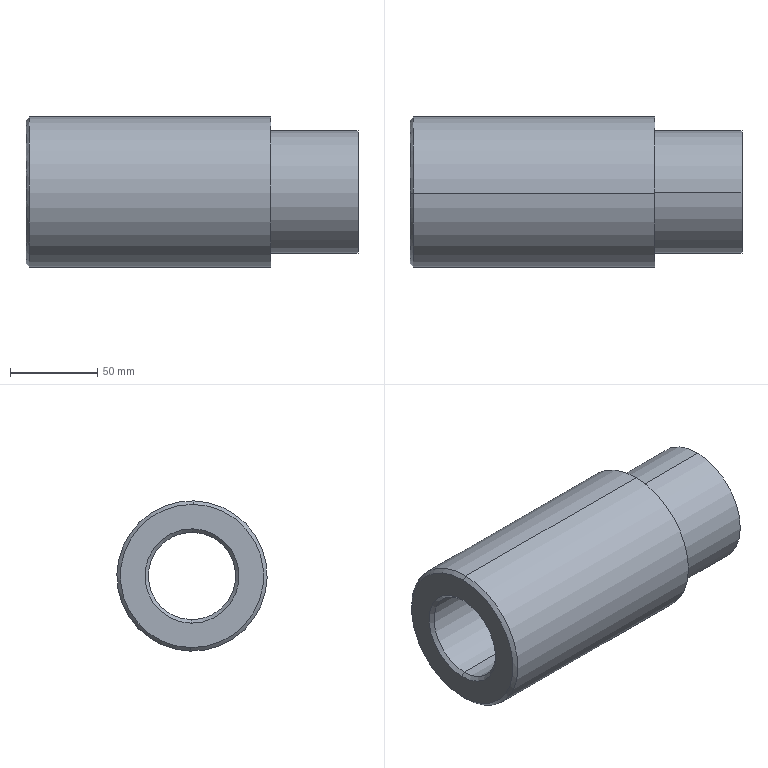Component | SolidWorks | 216InnerTubeAssembly-1_SpringSleeve-1 | 1 solid | 18 faces | box 190 x 86 x 86 mm | volume 501706 mm3 | cylinder 8 | cone 6 | plane 4 | commonest cylinder face diameters 86 x2 69.99 x2 60 x2 50 x2 | material Alloy Steel
build123d program:
from build123d import *


with BuildPart() as part:
    # Model → Revolve1 (revolve)
    with BuildSketch(Plane.XY, mode=Mode.PRIVATE) as revolve1_sk:
        Polygon((-150.007, 25), (-188.007, 25), (-190.007, 27), (-190.007, 41), (-188.007, 43), (-50.007, 43), (-50.007, 34.995), (-0.006987, 34.995), (-0.006987, 32), (-2.007, 30), (-150.007, 30), align=None)
    revolve(revolve1_sk.sketch.rotate(Axis((0, 0, 0), (-1, 0, 0)), 90), axis=Axis((0, 0, 0), (-1, 0, 0)))


solid = part.part

# Placed as in the assembly
solid = solid.moved(Location((322.098, 0, 0), (0, 0, 0)))
STEP:
#1=CARTESIAN_POINT('',(5.279,-0.01767,0.9841));
#2=VERTEX_POINT('',#1);
#3=CARTESIAN_POINT('',(5.279,0.01767,-0.9841));
#4=VERTEX_POINT('',#3);
#5=CARTESIAN_POINT('',(5.279,-0.,0.));
#6=DIRECTION('',(1.,0.,-0.));
#7=DIRECTION('',(0.,0.01796,-0.9998));
#8=AXIS2_PLACEMENT_3D('',#5,#6,#7);
#9=CIRCLE('',#8,0.9843);
#10=EDGE_CURVE('',#2,#4,#9,.T.);
#11=ORIENTED_EDGE('',*,*,#10,.T.);
#12=CARTESIAN_POINT('',(5.2,0.01909,-1.063));
#13=VERTEX_POINT('',#12);
#14=CARTESIAN_POINT('',(5.279,0.01767,-0.9841));
#15=DIRECTION('',(-0.7071,0.0127,-0.707));
#16=VECTOR('',#15,39.37);
#17=LINE('',#14,#16);
#18=EDGE_CURVE('',#4,#13,#17,.T.);
#19=ORIENTED_EDGE('',*,*,#18,.T.);
#20=CARTESIAN_POINT('',(5.2,-0.01909,1.063));
#21=VERTEX_POINT('',#20);
#22=CARTESIAN_POINT('',(5.2,-0.,0.));
#23=DIRECTION('',(1.,0.,-0.));
#24=DIRECTION('',(0.,0.01796,-0.9998));
#25=AXIS2_PLACEMENT_3D('',#22,#23,#24);
#26=CIRCLE('',#25,1.063);
#27=EDGE_CURVE('',#21,#13,#26,.T.);
#28=ORIENTED_EDGE('',*,*,#27,.F.);
#29=CARTESIAN_POINT('',(5.279,-0.01767,0.9841));
#30=DIRECTION('',(-0.7071,-0.0127,0.707));
#31=VECTOR('',#30,39.37);
#32=LINE('',#29,#31);
#33=EDGE_CURVE('',#2,#21,#32,.T.);
#34=ORIENTED_EDGE('',*,*,#33,.F.);
#35=EDGE_LOOP('',(#11,#19,#28,#34));
#36=FACE_OUTER_BOUND('',#35,.T.);
#37=CARTESIAN_POINT('',(5.279,-0.,0.));
#38=DIRECTION('',(-1.,-0.,0.));
#39=DIRECTION('',(0.,-0.01796,0.9998));
#40=AXIS2_PLACEMENT_3D('',#37,#38,#39);
#41=CONICAL_SURFACE('',#40,0.9843,0.7854);
#42=ADVANCED_FACE('',(#36),#41,.F.);
#43=CARTESIAN_POINT('',(5.2,0.02898,-1.614));
#44=VERTEX_POINT('',#43);
#45=CARTESIAN_POINT('',(5.2,-0.02898,1.614));
#46=VERTEX_POINT('',#45);
#47=CARTESIAN_POINT('',(5.2,-0.,0.));
#48=DIRECTION('',(1.,0.,-0.));
#49=DIRECTION('',(0.,0.01796,-0.9998));
#50=AXIS2_PLACEMENT_3D('',#47,#48,#49);
#51=CIRCLE('',#50,1.614);
#52=EDGE_CURVE('',#44,#46,#51,.T.);
#53=ORIENTED_EDGE('',*,*,#52,.T.);
#54=CARTESIAN_POINT('',(5.279,-0.0304,1.693));
#55=VERTEX_POINT('',#54);
#56=CARTESIAN_POINT('',(5.279,-0.0304,1.693));
#57=DIRECTION('',(0.7071,-0.0127,0.707));
#58=VECTOR('',#57,39.37);
#59=LINE('',#56,#58);
#60=EDGE_CURVE('',#46,#55,#59,.T.);
#61=ORIENTED_EDGE('',*,*,#60,.T.);
#62=CARTESIAN_POINT('',(5.279,0.0304,-1.693));
#63=VERTEX_POINT('',#62);
#64=CARTESIAN_POINT('',(5.279,-0.,0.));
#65=DIRECTION('',(1.,0.,-0.));
#66=DIRECTION('',(0.,0.01796,-0.9998));
#67=AXIS2_PLACEMENT_3D('',#64,#65,#66);
#68=CIRCLE('',#67,1.693);
#69=EDGE_CURVE('',#63,#55,#68,.T.);
#70=ORIENTED_EDGE('',*,*,#69,.F.);
#71=CARTESIAN_POINT('',(5.279,0.0304,-1.693));
#72=DIRECTION('',(0.7071,0.0127,-0.707));
#73=VECTOR('',#72,39.37);
#74=LINE('',#71,#73);
#75=EDGE_CURVE('',#44,#63,#74,.T.);
#76=ORIENTED_EDGE('',*,*,#75,.F.);
#77=EDGE_LOOP('',(#53,#61,#70,#76));
#78=FACE_OUTER_BOUND('',#77,.T.);
#79=CARTESIAN_POINT('',(5.279,-0.,0.));
#80=DIRECTION('',(1.,0.,-0.));
#81=DIRECTION('',(0.,0.01796,-0.9998));
#82=AXIS2_PLACEMENT_3D('',#79,#80,#81);
#83=CONICAL_SURFACE('',#82,1.693,0.7854);
#84=ADVANCED_FACE('',(#78),#83,.T.);
#85=ORIENTED_EDGE('',*,*,#69,.T.);
#86=CARTESIAN_POINT('',(10.712,-0.0304,1.693));
#87=VERTEX_POINT('',#86);
#88=CARTESIAN_POINT('',(12.681,-0.0304,1.693));
#89=DIRECTION('',(1.,0.,-0.));
#90=VECTOR('',#89,39.37);
#91=LINE('',#88,#90);
#92=EDGE_CURVE('',#55,#87,#91,.T.);
#93=ORIENTED_EDGE('',*,*,#92,.T.);
#94=CARTESIAN_POINT('',(10.712,0.0304,-1.693));
#95=VERTEX_POINT('',#94);
#96=CARTESIAN_POINT('',(10.712,-0.,0.));
#97=DIRECTION('',(1.,0.,-0.));
#98=DIRECTION('',(0.,0.01796,-0.9998));
#99=AXIS2_PLACEMENT_3D('',#96,#97,#98);
#100=CIRCLE('',#99,1.693);
#101=EDGE_CURVE('',#95,#87,#100,.T.);
#102=ORIENTED_EDGE('',*,*,#101,.F.);
#103=CARTESIAN_POINT('',(12.681,0.0304,-1.693));
#104=DIRECTION('',(1.,0.,-0.));
#105=VECTOR('',#104,39.37);
#106=LINE('',#103,#105);
#107=EDGE_CURVE('',#63,#95,#106,.T.);
#108=ORIENTED_EDGE('',*,*,#107,.F.);
#109=EDGE_LOOP('',(#85,#93,#102,#108));
#110=FACE_OUTER_BOUND('',#109,.T.);
#111=CARTESIAN_POINT('',(12.681,-0.,0.));
#112=DIRECTION('',(1.,0.,-0.));
#113=DIRECTION('',(0.,0.01796,-0.9998));
#114=AXIS2_PLACEMENT_3D('',#111,#112,#113);
#115=CYLINDRICAL_SURFACE('',#114,1.693);
#116=ADVANCED_FACE('',(#110),#115,.T.);
#117=CARTESIAN_POINT('',(10.712,0.02474,-1.378));
#118=VERTEX_POINT('',#117);
#119=CARTESIAN_POINT('',(10.712,-0.02474,1.378));
#120=VERTEX_POINT('',#119);
#121=CARTESIAN_POINT('',(10.712,-0.,0.));
#122=DIRECTION('',(1.,0.,-0.));
#123=DIRECTION('',(0.,0.01796,-0.9998));
#124=AXIS2_PLACEMENT_3D('',#121,#122,#123);
#125=CIRCLE('',#124,1.378);
#126=EDGE_CURVE('',#118,#120,#125,.T.);
#127=ORIENTED_EDGE('',*,*,#126,.T.);
#128=CARTESIAN_POINT('',(12.681,-0.02474,1.378));
#129=VERTEX_POINT('',#128);
#130=CARTESIAN_POINT('',(12.681,-0.02474,1.378));
#131=DIRECTION('',(1.,0.,-0.));
#132=VECTOR('',#131,39.37);
#133=LINE('',#130,#132);
#134=EDGE_CURVE('',#120,#129,#133,.T.);
#135=ORIENTED_EDGE('',*,*,#134,.T.);
#136=CARTESIAN_POINT('',(12.681,0.02474,-1.378));
#137=VERTEX_POINT('',#136);
#138=CARTESIAN_POINT('',(12.681,-0.,0.));
#139=DIRECTION('',(1.,0.,-0.));
#140=DIRECTION('',(0.,0.01796,-0.9998));
#141=AXIS2_PLACEMENT_3D('',#138,#139,#140);
#142=CIRCLE('',#141,1.378);
#143=EDGE_CURVE('',#137,#129,#142,.T.);
#144=ORIENTED_EDGE('',*,*,#143,.F.);
#145=CARTESIAN_POINT('',(12.681,0.02474,-1.378));
#146=DIRECTION('',(1.,0.,-0.));
#147=VECTOR('',#146,39.37);
#148=LINE('',#145,#147);
#149=EDGE_CURVE('',#118,#137,#148,.T.);
#150=ORIENTED_EDGE('',*,*,#149,.F.);
#151=EDGE_LOOP('',(#127,#135,#144,#150));
#152=FACE_OUTER_BOUND('',#151,.T.);
#153=CARTESIAN_POINT('',(12.681,-0.,0.));
#154=DIRECTION('',(1.,0.,-0.));
#155=DIRECTION('',(0.,0.01796,-0.9998));
#156=AXIS2_PLACEMENT_3D('',#153,#154,#155);
#157=CYLINDRICAL_SURFACE('',#156,1.378);
#158=ADVANCED_FACE('',(#152),#157,.T.);
#159=CARTESIAN_POINT('',(12.602,-0.02121,1.181));
#160=VERTEX_POINT('',#159);
#161=CARTESIAN_POINT('',(12.602,0.02121,-1.181));
#162=VERTEX_POINT('',#161);
#163=CARTESIAN_POINT('',(12.602,-0.,0.));
#164=DIRECTION('',(1.,0.,-0.));
#165=DIRECTION('',(0.,0.01796,-0.9998));
#166=AXIS2_PLACEMENT_3D('',#163,#164,#165);
#167=CIRCLE('',#166,1.181);
#168=EDGE_CURVE('',#160,#162,#167,.T.);
#169=ORIENTED_EDGE('',*,*,#168,.F.);
#170=CARTESIAN_POINT('',(12.681,-0.02262,1.26));
#171=VERTEX_POINT('',#170);
#172=CARTESIAN_POINT('',(12.681,-0.02262,1.26));
#173=DIRECTION('',(0.7071,-0.0127,0.707));
#174=VECTOR('',#173,39.37);
#175=LINE('',#172,#174);
#176=EDGE_CURVE('',#160,#171,#175,.T.);
#177=ORIENTED_EDGE('',*,*,#176,.T.);
#178=CARTESIAN_POINT('',(12.681,0.02262,-1.26));
#179=VERTEX_POINT('',#178);
#180=CARTESIAN_POINT('',(12.681,-0.,0.));
#181=DIRECTION('',(1.,0.,-0.));
#182=DIRECTION('',(0.,0.01796,-0.9998));
#183=AXIS2_PLACEMENT_3D('',#180,#181,#182);
#184=CIRCLE('',#183,1.26);
#185=EDGE_CURVE('',#171,#179,#184,.T.);
#186=ORIENTED_EDGE('',*,*,#185,.T.);
#187=CARTESIAN_POINT('',(12.681,0.02262,-1.26));
#188=DIRECTION('',(0.7071,0.0127,-0.707));
#189=VECTOR('',#188,39.37);
#190=LINE('',#187,#189);
#191=EDGE_CURVE('',#162,#179,#190,.T.);
#192=ORIENTED_EDGE('',*,*,#191,.F.);
#193=EDGE_LOOP('',(#169,#177,#186,#192));
#194=FACE_OUTER_BOUND('',#193,.T.);
#195=CARTESIAN_POINT('',(12.681,-0.,0.));
#196=DIRECTION('',(1.,0.,-0.));
#197=DIRECTION('',(0.,0.01796,-0.9998));
#198=AXIS2_PLACEMENT_3D('',#195,#196,#197);
#199=CONICAL_SURFACE('',#198,1.26,0.7854);
#200=ADVANCED_FACE('',(#194),#199,.F.);
#201=CARTESIAN_POINT('',(6.775,-0.02121,1.181));
#202=VERTEX_POINT('',#201);
#203=CARTESIAN_POINT('',(6.775,0.02121,-1.181));
#204=VERTEX_POINT('',#203);
#205=CARTESIAN_POINT('',(6.775,-0.,0.));
#206=DIRECTION('',(1.,0.,-0.));
#207=DIRECTION('',(0.,0.01796,-0.9998));
#208=AXIS2_PLACEMENT_3D('',#205,#206,#207);
#209=CIRCLE('',#208,1.181);
#210=EDGE_CURVE('',#202,#204,#209,.T.);
#211=ORIENTED_EDGE('',*,*,#210,.F.);
#212=CARTESIAN_POINT('',(12.681,-0.02121,1.181));
#213=DIRECTION('',(1.,0.,-0.));
#214=VECTOR('',#213,39.37);
#215=LINE('',#212,#214);
#216=EDGE_CURVE('',#202,#160,#215,.T.);
#217=ORIENTED_EDGE('',*,*,#216,.T.);
#218=ORIENTED_EDGE('',*,*,#168,.T.);
#219=CARTESIAN_POINT('',(12.681,0.02121,-1.181));
#220=DIRECTION('',(1.,0.,-0.));
#221=VECTOR('',#220,39.37);
#222=LINE('',#219,#221);
#223=EDGE_CURVE('',#204,#162,#222,.T.);
#224=ORIENTED_EDGE('',*,*,#223,.F.);
#225=EDGE_LOOP('',(#211,#217,#218,#224));
#226=FACE_OUTER_BOUND('',#225,.T.);
#227=CARTESIAN_POINT('',(12.681,-0.,0.));
#228=DIRECTION('',(1.,0.,-0.));
#229=DIRECTION('',(0.,0.01796,-0.9998));
#230=AXIS2_PLACEMENT_3D('',#227,#228,#229);
#231=CYLINDRICAL_SURFACE('',#230,1.181);
#232=ADVANCED_FACE('',(#226),#231,.F.);
#233=ORIENTED_EDGE('',*,*,#10,.F.);
#234=CARTESIAN_POINT('',(6.775,-0.01767,0.9841));
#235=VERTEX_POINT('',#234);
#236=CARTESIAN_POINT('',(12.681,-0.01767,0.9841));
#237=DIRECTION('',(1.,0.,-0.));
#238=VECTOR('',#237,39.37);
#239=LINE('',#236,#238);
#240=EDGE_CURVE('',#2,#235,#239,.T.);
#241=ORIENTED_EDGE('',*,*,#240,.T.);
#242=CARTESIAN_POINT('',(6.775,0.01767,-0.9841));
#243=VERTEX_POINT('',#242);
#244=CARTESIAN_POINT('',(6.775,-0.,0.));
#245=DIRECTION('',(1.,0.,-0.));
#246=DIRECTION('',(0.,0.01796,-0.9998));
#247=AXIS2_PLACEMENT_3D('',#244,#245,#246);
#248=CIRCLE('',#247,0.9843);
#249=EDGE_CURVE('',#235,#243,#248,.T.);
#250=ORIENTED_EDGE('',*,*,#249,.T.);
#251=CARTESIAN_POINT('',(12.681,0.01767,-0.9841));
#252=DIRECTION('',(1.,0.,-0.));
#253=VECTOR('',#252,39.37);
#254=LINE('',#251,#253);
#255=EDGE_CURVE('',#4,#243,#254,.T.);
#256=ORIENTED_EDGE('',*,*,#255,.F.);
#257=EDGE_LOOP('',(#233,#241,#250,#256));
#258=FACE_OUTER_BOUND('',#257,.T.);
#259=CARTESIAN_POINT('',(12.681,-0.,0.));
#260=DIRECTION('',(1.,0.,-0.));
#261=DIRECTION('',(0.,0.01796,-0.9998));
#262=AXIS2_PLACEMENT_3D('',#259,#260,#261);
#263=CYLINDRICAL_SURFACE('',#262,0.9843);
#264=ADVANCED_FACE('',(#258),#263,.F.);
#265=ORIENTED_EDGE('',*,*,#240,.F.);
#266=CARTESIAN_POINT('',(5.279,-0.,0.));
#267=DIRECTION('',(1.,0.,-0.));
#268=DIRECTION('',(0.,0.01796,-0.9998));
#269=AXIS2_PLACEMENT_3D('',#266,#267,#268);
#270=CIRCLE('',#269,0.9843);
#271=EDGE_CURVE('',#4,#2,#270,.T.);
#272=ORIENTED_EDGE('',*,*,#271,.F.);
#273=ORIENTED_EDGE('',*,*,#255,.T.);
#274=CARTESIAN_POINT('',(6.775,-0.,0.));
#275=DIRECTION('',(1.,0.,-0.));
#276=DIRECTION('',(0.,0.01796,-0.9998));
#277=AXIS2_PLACEMENT_3D('',#274,#275,#276);
#278=CIRCLE('',#277,0.9843);
#279=EDGE_CURVE('',#243,#235,#278,.T.);
#280=ORIENTED_EDGE('',*,*,#279,.T.);
#281=EDGE_LOOP('',(#265,#272,#273,#280));
#282=FACE_OUTER_BOUND('',#281,.T.);
#283=CARTESIAN_POINT('',(12.681,-0.,0.));
#284=DIRECTION('',(1.,0.,-0.));
#285=DIRECTION('',(0.,0.01796,-0.9998));
#286=AXIS2_PLACEMENT_3D('',#283,#284,#285);
#287=CYLINDRICAL_SURFACE('',#286,0.9843);
#288=ADVANCED_FACE('',(#282),#287,.F.);
#289=CARTESIAN_POINT('',(6.775,-0.,0.));
#290=DIRECTION('',(1.,0.,-0.));
#291=DIRECTION('',(0.,0.01796,-0.9998));
#292=AXIS2_PLACEMENT_3D('',#289,#290,#291);
#293=CIRCLE('',#292,1.181);
#294=EDGE_CURVE('',#204,#202,#293,.T.);
#295=ORIENTED_EDGE('',*,*,#294,.T.);
#296=ORIENTED_EDGE('',*,*,#210,.T.);
#297=EDGE_LOOP('',(#295,#296));
#298=FACE_OUTER_BOUND('',#297,.T.);
#299=ORIENTED_EDGE('',*,*,#279,.F.);
#300=ORIENTED_EDGE('',*,*,#249,.F.);
#301=EDGE_LOOP('',(#299,#300));
#302=FACE_BOUND('',#301,.T.);
#303=CARTESIAN_POINT('',(6.775,-0.,0.));
#304=DIRECTION('',(1.,0.,-0.));
#305=DIRECTION('',(-0.,0.01796,-0.9998));
#306=AXIS2_PLACEMENT_3D('',#303,#304,#305);
#307=PLANE('',#306);
#308=ADVANCED_FACE('',(#298,#302),#307,.T.);
#309=ORIENTED_EDGE('',*,*,#216,.F.);
#310=ORIENTED_EDGE('',*,*,#294,.F.);
#311=ORIENTED_EDGE('',*,*,#223,.T.);
#312=CARTESIAN_POINT('',(12.602,-0.,0.));
#313=DIRECTION('',(1.,0.,-0.));
#314=DIRECTION('',(0.,0.01796,-0.9998));
#315=AXIS2_PLACEMENT_3D('',#312,#313,#314);
#316=CIRCLE('',#315,1.181);
#317=EDGE_CURVE('',#162,#160,#316,.T.);
#318=ORIENTED_EDGE('',*,*,#317,.T.);
#319=EDGE_LOOP('',(#309,#310,#311,#318));
#320=FACE_OUTER_BOUND('',#319,.T.);
#321=CARTESIAN_POINT('',(12.681,-0.,0.));
#322=DIRECTION('',(1.,0.,-0.));
#323=DIRECTION('',(0.,0.01796,-0.9998));
#324=AXIS2_PLACEMENT_3D('',#321,#322,#323);
#325=CYLINDRICAL_SURFACE('',#324,1.181);
#326=ADVANCED_FACE('',(#320),#325,.F.);
#327=ORIENTED_EDGE('',*,*,#176,.F.);
#328=ORIENTED_EDGE('',*,*,#317,.F.);
#329=ORIENTED_EDGE('',*,*,#191,.T.);
#330=CARTESIAN_POINT('',(12.681,-0.,0.));
#331=DIRECTION('',(1.,0.,-0.));
#332=DIRECTION('',(0.,0.01796,-0.9998));
#333=AXIS2_PLACEMENT_3D('',#330,#331,#332);
#334=CIRCLE('',#333,1.26);
#335=EDGE_CURVE('',#179,#171,#334,.T.);
#336=ORIENTED_EDGE('',*,*,#335,.T.);
#337=EDGE_LOOP('',(#327,#328,#329,#336));
#338=FACE_OUTER_BOUND('',#337,.T.);
#339=CARTESIAN_POINT('',(12.681,-0.,0.));
#340=DIRECTION('',(1.,0.,-0.));
#341=DIRECTION('',(0.,0.01796,-0.9998));
#342=AXIS2_PLACEMENT_3D('',#339,#340,#341);
#343=CONICAL_SURFACE('',#342,1.26,0.7854);
#344=ADVANCED_FACE('',(#338),#343,.F.);
#345=ORIENTED_EDGE('',*,*,#335,.F.);
#346=ORIENTED_EDGE('',*,*,#185,.F.);
#347=EDGE_LOOP('',(#345,#346));
#348=FACE_BOUND('',#347,.T.);
#349=ORIENTED_EDGE('',*,*,#143,.T.);
#350=CARTESIAN_POINT('',(12.681,-0.,0.));
#351=DIRECTION('',(1.,0.,-0.));
#352=DIRECTION('',(0.,0.01796,-0.9998));
#353=AXIS2_PLACEMENT_3D('',#350,#351,#352);
#354=CIRCLE('',#353,1.378);
#355=EDGE_CURVE('',#129,#137,#354,.T.);
#356=ORIENTED_EDGE('',*,*,#355,.T.);
#357=EDGE_LOOP('',(#349,#356));
#358=FACE_OUTER_BOUND('',#357,.T.);
#359=CARTESIAN_POINT('',(12.681,-0.,0.));
#360=DIRECTION('',(-1.,-0.,0.));
#361=DIRECTION('',(0.,-0.01796,0.9998));
#362=AXIS2_PLACEMENT_3D('',#359,#360,#361);
#363=PLANE('',#362);
#364=ADVANCED_FACE('',(#348,#358),#363,.F.);
#365=ORIENTED_EDGE('',*,*,#134,.F.);
#366=CARTESIAN_POINT('',(10.712,-0.,0.));
#367=DIRECTION('',(1.,0.,-0.));
#368=DIRECTION('',(0.,0.01796,-0.9998));
#369=AXIS2_PLACEMENT_3D('',#366,#367,#368);
#370=CIRCLE('',#369,1.378);
#371=EDGE_CURVE('',#120,#118,#370,.T.);
#372=ORIENTED_EDGE('',*,*,#371,.T.);
#373=ORIENTED_EDGE('',*,*,#149,.T.);
#374=ORIENTED_EDGE('',*,*,#355,.F.);
#375=EDGE_LOOP('',(#365,#372,#373,#374));
#376=FACE_OUTER_BOUND('',#375,.T.);
#377=CARTESIAN_POINT('',(12.681,-0.,0.));
#378=DIRECTION('',(1.,0.,-0.));
#379=DIRECTION('',(0.,0.01796,-0.9998));
#380=AXIS2_PLACEMENT_3D('',#377,#378,#379);
#381=CYLINDRICAL_SURFACE('',#380,1.378);
#382=ADVANCED_FACE('',(#376),#381,.T.);
#383=ORIENTED_EDGE('',*,*,#101,.T.);
#384=CARTESIAN_POINT('',(10.712,-0.,0.));
#385=DIRECTION('',(1.,0.,-0.));
#386=DIRECTION('',(0.,0.01796,-0.9998));
#387=AXIS2_PLACEMENT_3D('',#384,#385,#386);
#388=CIRCLE('',#387,1.693);
#389=EDGE_CURVE('',#87,#95,#388,.T.);
#390=ORIENTED_EDGE('',*,*,#389,.T.);
#391=EDGE_LOOP('',(#383,#390));
#392=FACE_OUTER_BOUND('',#391,.T.);
#393=ORIENTED_EDGE('',*,*,#126,.F.);
#394=ORIENTED_EDGE('',*,*,#371,.F.);
#395=EDGE_LOOP('',(#393,#394));
#396=FACE_BOUND('',#395,.T.);
#397=CARTESIAN_POINT('',(10.712,-0.,0.));
#398=DIRECTION('',(1.,0.,-0.));
#399=DIRECTION('',(-0.,0.01796,-0.9998));
#400=AXIS2_PLACEMENT_3D('',#397,#398,#399);
#401=PLANE('',#400);
#402=ADVANCED_FACE('',(#392,#396),#401,.T.);
#403=ORIENTED_EDGE('',*,*,#92,.F.);
#404=CARTESIAN_POINT('',(5.279,-0.,0.));
#405=DIRECTION('',(1.,0.,-0.));
#406=DIRECTION('',(0.,0.01796,-0.9998));
#407=AXIS2_PLACEMENT_3D('',#404,#405,#406);
#408=CIRCLE('',#407,1.693);
#409=EDGE_CURVE('',#55,#63,#408,.T.);
#410=ORIENTED_EDGE('',*,*,#409,.T.);
#411=ORIENTED_EDGE('',*,*,#107,.T.);
#412=ORIENTED_EDGE('',*,*,#389,.F.);
#413=EDGE_LOOP('',(#403,#410,#411,#412));
#414=FACE_OUTER_BOUND('',#413,.T.);
#415=CARTESIAN_POINT('',(12.681,-0.,0.));
#416=DIRECTION('',(1.,0.,-0.));
#417=DIRECTION('',(0.,0.01796,-0.9998));
#418=AXIS2_PLACEMENT_3D('',#415,#416,#417);
#419=CYLINDRICAL_SURFACE('',#418,1.693);
#420=ADVANCED_FACE('',(#414),#419,.T.);
#421=ORIENTED_EDGE('',*,*,#60,.F.);
#422=CARTESIAN_POINT('',(5.2,-0.,0.));
#423=DIRECTION('',(1.,0.,-0.));
#424=DIRECTION('',(0.,0.01796,-0.9998));
#425=AXIS2_PLACEMENT_3D('',#422,#423,#424);
#426=CIRCLE('',#425,1.614);
#427=EDGE_CURVE('',#46,#44,#426,.T.);
#428=ORIENTED_EDGE('',*,*,#427,.T.);
#429=ORIENTED_EDGE('',*,*,#75,.T.);
#430=ORIENTED_EDGE('',*,*,#409,.F.);
#431=EDGE_LOOP('',(#421,#428,#429,#430));
#432=FACE_OUTER_BOUND('',#431,.T.);
#433=CARTESIAN_POINT('',(5.279,-0.,0.));
#434=DIRECTION('',(1.,0.,-0.));
#435=DIRECTION('',(0.,0.01796,-0.9998));
#436=AXIS2_PLACEMENT_3D('',#433,#434,#435);
#437=CONICAL_SURFACE('',#436,1.693,0.7854);
#438=ADVANCED_FACE('',(#432),#437,.T.);
#439=ORIENTED_EDGE('',*,*,#27,.T.);
#440=CARTESIAN_POINT('',(5.2,-0.,0.));
#441=DIRECTION('',(1.,0.,-0.));
#442=DIRECTION('',(0.,0.01796,-0.9998));
#443=AXIS2_PLACEMENT_3D('',#440,#441,#442);
#444=CIRCLE('',#443,1.063);
#445=EDGE_CURVE('',#13,#21,#444,.T.);
#446=ORIENTED_EDGE('',*,*,#445,.T.);
#447=EDGE_LOOP('',(#439,#446));
#448=FACE_BOUND('',#447,.T.);
#449=ORIENTED_EDGE('',*,*,#52,.F.);
#450=ORIENTED_EDGE('',*,*,#427,.F.);
#451=EDGE_LOOP('',(#449,#450));
#452=FACE_OUTER_BOUND('',#451,.T.);
#453=CARTESIAN_POINT('',(5.2,-0.,0.));
#454=DIRECTION('',(-1.,-0.,0.));
#455=DIRECTION('',(0.,-0.01796,0.9998));
#456=AXIS2_PLACEMENT_3D('',#453,#454,#455);
#457=PLANE('',#456);
#458=ADVANCED_FACE('',(#448,#452),#457,.T.);
#459=ORIENTED_EDGE('',*,*,#18,.F.);
#460=ORIENTED_EDGE('',*,*,#271,.T.);
#461=ORIENTED_EDGE('',*,*,#33,.T.);
#462=ORIENTED_EDGE('',*,*,#445,.F.);
#463=EDGE_LOOP('',(#459,#460,#461,#462));
#464=FACE_OUTER_BOUND('',#463,.T.);
#465=CARTESIAN_POINT('',(5.279,-0.,0.));
#466=DIRECTION('',(-1.,-0.,0.));
#467=DIRECTION('',(0.,-0.01796,0.9998));
#468=AXIS2_PLACEMENT_3D('',#465,#466,#467);
#469=CONICAL_SURFACE('',#468,0.9843,0.7854);
#470=ADVANCED_FACE('',(#464),#469,.F.);
#471=CLOSED_SHELL('',(#42,#84,#116,#158,#200,#232,#264,#288,#308,#326,#344,#364,#382,#402,#420,#438,#458,#470));
#472=MANIFOLD_SOLID_BREP('',#471);
#473=CARTESIAN_POINT('',(0.,0.,0.));
#474=DIRECTION('',(0.,0.,1.));
#475=DIRECTION('',(1.,0.,0.));
#476=AXIS2_PLACEMENT_3D('',#473,#474,#475);
#477=(LENGTH_UNIT()NAMED_UNIT(*)SI_UNIT($,.METRE.));
#478=LENGTH_MEASURE_WITH_UNIT(LENGTH_MEASURE(0.0254),#477);
#479=DIMENSIONAL_EXPONENTS(1.,0.,0.,0.,0.,0.,0.);
#480=(CONVERSION_BASED_UNIT('',#478)LENGTH_UNIT()NAMED_UNIT(#479));
#481=UNCERTAINTY_MEASURE_WITH_UNIT(LENGTH_MEASURE(0.00001),#480,'','');
#482=(NAMED_UNIT(*)PLANE_ANGLE_UNIT()SI_UNIT($,.RADIAN.));
#483=(NAMED_UNIT(*)SI_UNIT($,.STERADIAN.)SOLID_ANGLE_UNIT());
#484=(GEOMETRIC_REPRESENTATION_CONTEXT(3)GLOBAL_UNCERTAINTY_ASSIGNED_CONTEXT((#481))GLOBAL_UNIT_ASSIGNED_CONTEXT((#480,#482,#483))REPRESENTATION_CONTEXT('',''));
#485=ADVANCED_BREP_SHAPE_REPRESENTATION('',(#472,#476),#484);
#486=COLOUR_RGB('',0.7922,0.8196,0.9333);
#487=FILL_AREA_STYLE_COLOUR('',#486);
#488=FILL_AREA_STYLE('',(#487));
#489=SURFACE_STYLE_FILL_AREA(#488);
#490=SURFACE_SIDE_STYLE('',(#489));
#491=SURFACE_STYLE_USAGE(.BOTH.,#490);
#492=PRESENTATION_STYLE_ASSIGNMENT((#491));
#493=STYLED_ITEM('',(#492),#472);
#494=(LENGTH_UNIT()NAMED_UNIT(*)SI_UNIT($,.METRE.));
#495=LENGTH_MEASURE_WITH_UNIT(LENGTH_MEASURE(0.0254),#494);
#496=DIMENSIONAL_EXPONENTS(1.,0.,0.,0.,0.,0.,0.);
#497=(CONVERSION_BASED_UNIT('',#495)LENGTH_UNIT()NAMED_UNIT(#496));
#498=UNCERTAINTY_MEASURE_WITH_UNIT(LENGTH_MEASURE(0.00001),#497,'','');
#499=(NAMED_UNIT(*)PLANE_ANGLE_UNIT()SI_UNIT($,.RADIAN.));
#500=(NAMED_UNIT(*)SI_UNIT($,.STERADIAN.)SOLID_ANGLE_UNIT());
#501=(GEOMETRIC_REPRESENTATION_CONTEXT(3)GLOBAL_UNCERTAINTY_ASSIGNED_CONTEXT((#498))GLOBAL_UNIT_ASSIGNED_CONTEXT((#497,#499,#500))REPRESENTATION_CONTEXT('',''));
#502=MECHANICAL_DESIGN_GEOMETRIC_PRESENTATION_REPRESENTATION('',(#493),#501);
#503=PRESENTATION_LAYER_ASSIGNMENT('','',(#493));